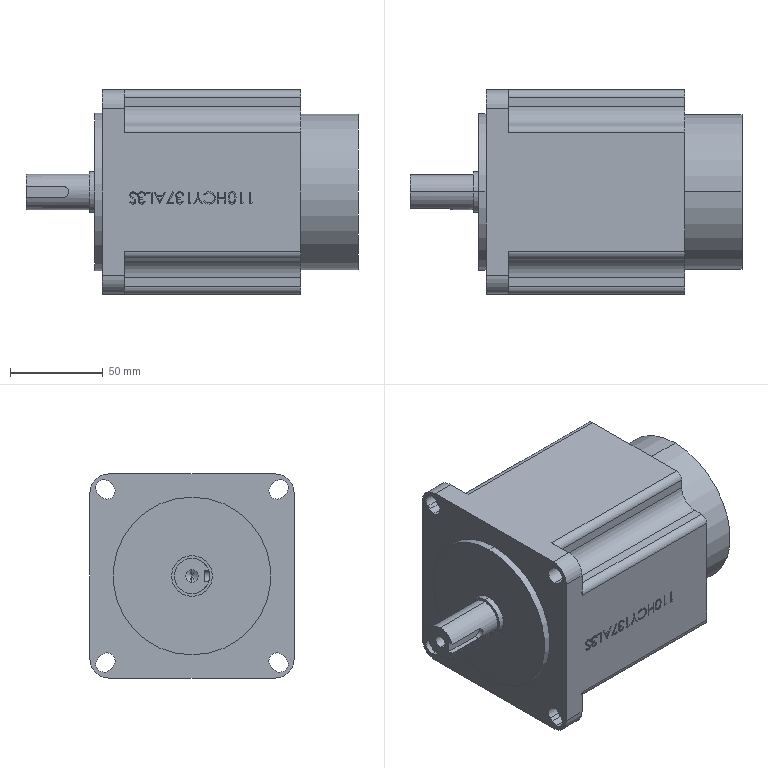Component | SolidWorks | ElectricalBoxAssembly2-1_StepperMotor-1 | 1 solid | 222 faces | box 179 x 110 x 110 mm | volume 1361866 mm3 | plane 120 | spline 61 | cylinder 39 | cone 2 | commonest cylinder face diameters 9 x12 20 x8 8 x8 6.8 x2 19 x2 22 x2 84 x2 85 x2
build123d program:
from build123d import *

# Parameters (mm, degrees)
SKETCH1_W             = 110
SKETCH1_H             = 110
BOSS_EXTRUDE1_DEPTH   = 12
SKETCH3_R             = 42.5
BOSS_EXTRUDE2_DEPTH   = 4
SKETCH4_R             = 9.5
BOSS_EXTRUDE3_DEPTH   = 37
CUT_EXTRUDE1_DEPTH    = 88.926
BOSS_EXTRUDE4_DEPTH   = 95
FILLET1_R             = 10
CUT_EXTRUDE2_DEPTH    = 3
SKETCH9_R             = 42
BOSS_EXTRUDE5_DEPTH   = 31
CUT_EXTRUDE3_DEPTH    = 0.1
SKETCH11_R            = 11
BOSS_EXTRUDE6_DEPTH   = 3
M8_TAPPED_HOLE1_D     = 6.8
M8_TAPPED_HOLE1_DEPTH = 15.4
M8_TAPPED_HOLE1_TIP   = 2.043


with BuildPart() as part:
    # Sketch1 → Boss-Extrude1 (new body)
    with BuildSketch(Plane(origin=(0, 0, 0), x_dir=(0, 0, -1), z_dir=(1, 0, 0))):
        Rectangle(SKETCH1_W, SKETCH1_H)
    extrude(amount=BOSS_EXTRUDE1_DEPTH)

    # Sketch3 → Boss-Extrude2 (add)
    with BuildSketch(Plane(origin=(12, 0, 0), x_dir=(0, 0, -1), z_dir=(1, 0, 0))):
        Circle(SKETCH3_R)
    extrude(amount=BOSS_EXTRUDE2_DEPTH)

    # Sketch4 → Boss-Extrude3 (add)
    with BuildSketch(Plane(origin=(16, 0, 0), x_dir=(0, 0, -1), z_dir=(1, 0, 0))):
        Circle(SKETCH4_R)
    extrude(amount=BOSS_EXTRUDE3_DEPTH)

    # Sketch5 → Cut-Extrude1 (cut, through all)
    with BuildSketch(Plane(origin=(12, 0, 0), x_dir=(0, 0, -1), z_dir=(1, 0, 0))):
        with BuildLine():
            Line((-44.194, 50.558), (-42.78, 49.144))
            ThreePointArc((-42.78, 49.144), (-42.78, 42.78), (-49.144, 42.78))
            Line((-49.144, 42.78), (-50.558, 44.194))
            ThreePointArc((-50.558, 44.194), (-50.558, 50.558), (-44.194, 50.558))
        make_face()
        with BuildLine():
            Line((50.558, 44.194), (49.144, 42.78))
            ThreePointArc((49.144, 42.78), (42.78, 42.78), (42.78, 49.144))
            Line((42.78, 49.144), (44.194, 50.558))
            ThreePointArc((44.194, 50.558), (50.558, 50.558), (50.558, 44.194))
        make_face()
        with BuildLine():
            Line((44.194, -50.558), (42.78, -49.144))
            ThreePointArc((42.78, -49.144), (42.78, -42.78), (49.144, -42.78))
            Line((49.144, -42.78), (50.558, -44.194))
            ThreePointArc((50.558, -44.194), (50.558, -50.558), (44.194, -50.558))
        make_face()
        with BuildLine():
            Line((-50.558, -44.194), (-49.144, -42.78))
            ThreePointArc((-49.144, -42.78), (-42.78, -42.78), (-42.78, -49.144))
            Line((-42.78, -49.144), (-44.194, -50.558))
            ThreePointArc((-44.194, -50.558), (-50.558, -50.558), (-50.558, -44.194))
        make_face()
    extrude(amount=-CUT_EXTRUDE1_DEPTH, mode=Mode.SUBTRACT)

    # Sketch6 → Boss-Extrude4 (add)
    with BuildSketch(Plane.ZY):
        with BuildLine():
            Line((31.962, -55), (-31.962, -55))
            ThreePointArc((-31.962, -55), (-34.79, -53.828), (-35.962, -51))
            Line((-35.962, -51), (-35.962, -45.962))
            ThreePointArc((-35.962, -45.962), (-38.891, -38.891), (-45.962, -35.962))
            Line((-45.962, -35.962), (-51, -35.962))
            ThreePointArc((-51, -35.962), (-53.828, -34.79), (-55, -31.962))
            Line((-55, -31.962), (-55, 31.962))
            ThreePointArc((-55, 31.962), (-53.828, 34.79), (-51, 35.962))
            Line((-51, 35.962), (-45.962, 35.962))
            ThreePointArc((-45.962, 35.962), (-38.891, 38.891), (-35.962, 45.962))
            Line((-35.962, 45.962), (-35.962, 51))
            ThreePointArc((-35.962, 51), (-34.79, 53.828), (-31.962, 55))
            Line((-31.962, 55), (31.962, 55))
            ThreePointArc((31.962, 55), (34.79, 53.828), (35.962, 51))
            Line((35.962, 51), (35.962, 45.962))
            ThreePointArc((35.962, 45.962), (38.891, 38.891), (45.962, 35.962))
            Line((45.962, 35.962), (51, 35.962))
            ThreePointArc((51, 35.962), (53.828, 34.79), (55, 31.962))
            Line((55, 31.962), (55, -31.962))
            ThreePointArc((55, -31.962), (53.828, -34.79), (51, -35.962))
            Line((51, -35.962), (45.962, -35.962))
            ThreePointArc((45.962, -35.962), (38.891, -38.891), (35.962, -45.962))
            Line((35.962, -45.962), (35.962, -51))
            ThreePointArc((35.962, -51), (34.79, -53.828), (31.962, -55))
        make_face()
    extrude(amount=BOSS_EXTRUDE4_DEPTH)

    # Fillet1
    fillet1_edges = [part.edges().sort_by_distance(p)[0] for p in [
        (6, -55, -55),
        (6, -55, 55),
        (6, 55, 55),
        (6, 55, -55),
    ]]
    fillet(fillet1_edges, radius=FILLET1_R)

    # Sketch7 → Cut-Extrude2 (cut)
    with BuildSketch(Plane(origin=(0, 9.5, 0), x_dir=(1, 0, 0), z_dir=(0, 1, 0))):
        with BuildLine():
            Line((73, -3), (33, -3))
            ThreePointArc((33, -3), (30, 0), (33, 3))
            Line((33, 3), (73, 3))
            ThreePointArc((73, 3), (76, 0), (73, -3))
        make_face()
    extrude(amount=-CUT_EXTRUDE2_DEPTH, mode=Mode.SUBTRACT)

    # Sketch9 → Boss-Extrude5 (add)
    with BuildSketch(Plane.ZY.offset(95)):
        Circle(SKETCH9_R)
    extrude(amount=BOSS_EXTRUDE5_DEPTH)

    # Sketch10 → Cut-Extrude3 (cut)
    # profile 1 of 13: a face of its own
    with BuildSketch(Plane(origin=(0, 55, 0), x_dir=(1, 0, 0), z_dir=(0, 1, 0))):
        Polygon((-68.662, 6.35), (-67.488, 6.35), (-67.488, 0), (-68.058, 0), (-68.058, 5.699), (-69.035, 5.699), align=None)
    # profile 2 of 13: a face of its own
    with BuildSketch(Plane(origin=(0, 55, 0), x_dir=(1, 0, 0), z_dir=(0, 1, 0))):
        Polygon((-63.778, 6.35), (-62.604, 6.35), (-62.604, 0), (-63.174, 0), (-63.174, 5.699), (-64.15, 5.699), align=None)
    # profile 3 of 13: a face of its own
    with BuildSketch(Plane(origin=(0, 55, 0), x_dir=(1, 0, 0), z_dir=(0, 1, 0))):
        with BuildLine():
            add(Edge.make_bspline(
                [(-60.243, 3.172), (-60.242, 3.274), (-60.241, 3.472), (-60.228, 3.76), (-60.207, 4.03), (-60.178, 4.283), (-60.142, 4.517), (-60.094, 4.734), (-60.04, 4.933), (-59.978, 5.115), (-59.907, 5.283), (-59.83, 5.44), (-59.744, 5.585), (-59.653, 5.721), (-59.554, 5.846), (-59.45, 5.962), (-59.337, 6.065), (-59.218, 6.159), (-59.093, 6.242), (-58.965, 6.314), (-58.833, 6.376), (-58.697, 6.425), (-58.557, 6.465), (-58.415, 6.493), (-58.269, 6.51), (-58.17, 6.512), (-58.12, 6.513)],
                knots=[0, 0, 0, 0, 1.646, 3.198, 4.664, 6.031, 7.308, 8.502, 9.612, 10.642, 11.616, 12.558, 13.465, 14.35, 15.204, 16.04, 16.86, 17.68, 18.487, 19.282, 20.062, 20.843, 21.62, 22.403, 23.19, 24, 24, 24, 24], degree=3))
            add(Edge.make_bspline(
                [(-58.12, 6.513), (-58.069, 6.512), (-57.969, 6.51), (-57.82, 6.493), (-57.675, 6.465), (-57.534, 6.425), (-57.396, 6.376), (-57.262, 6.314), (-57.131, 6.242), (-57.005, 6.158), (-56.883, 6.063), (-56.768, 5.957), (-56.66, 5.839), (-56.557, 5.711), (-56.463, 5.571), (-56.373, 5.421), (-56.292, 5.258), (-56.215, 5.085), (-56.148, 4.898), (-56.087, 4.697), (-56.039, 4.48), (-55.998, 4.248), (-55.966, 4.001), (-55.944, 3.738), (-55.931, 3.46), (-55.929, 3.27), (-55.928, 3.172)],
                knots=[0, 0, 0, 0, 0.8109, 1.613, 2.397, 3.182, 3.964, 4.75, 5.552, 6.362, 7.182, 8.026, 8.879, 9.751, 10.658, 11.592, 12.561, 13.573, 14.631, 15.753, 16.941, 18.2, 19.532, 20.947, 22.433, 24, 24, 24, 24], degree=3))
            add(Edge.make_bspline(
                [(-55.928, 3.172), (-55.929, 3.075), (-55.931, 2.886), (-55.943, 2.609), (-55.967, 2.348), (-55.996, 2.102), (-56.037, 1.871), (-56.087, 1.656), (-56.143, 1.455), (-56.211, 1.269), (-56.287, 1.097), (-56.368, 0.9359), (-56.456, 0.785), (-56.551, 0.6453), (-56.653, 0.5158), (-56.763, 0.3988), (-56.879, 0.2914), (-57.001, 0.1959), (-57.129, 0.1123), (-57.259, 0.03752), (-57.395, -0.02277), (-57.533, -0.07454), (-57.674, -0.1141), (-57.82, -0.1414), (-57.969, -0.1606), (-58.069, -0.1621), (-58.12, -0.1628)],
                knots=[0, 0, 0, 0, 1.562, 3.043, 4.452, 5.778, 7.032, 8.214, 9.334, 10.387, 11.391, 12.355, 13.287, 14.194, 15.073, 15.931, 16.776, 17.606, 18.423, 19.229, 20.022, 20.808, 21.593, 22.385, 23.188, 24, 24, 24, 24], degree=3))
            add(Edge.make_bspline(
                [(-58.12, -0.1628), (-58.17, -0.162), (-58.269, -0.1603), (-58.415, -0.143), (-58.557, -0.1153), (-58.695, -0.07644), (-58.831, -0.02888), (-58.962, 0.03309), (-59.089, 0.1044), (-59.213, 0.1857), (-59.331, 0.2788), (-59.444, 0.3818), (-59.548, 0.4973), (-59.646, 0.6233), (-59.738, 0.7588), (-59.823, 0.9056), (-59.902, 1.063), (-59.974, 1.233), (-60.038, 1.416), (-60.094, 1.616), (-60.138, 1.834), (-60.176, 2.068), (-60.207, 2.32), (-60.228, 2.589), (-60.241, 2.875), (-60.242, 3.072), (-60.243, 3.172)],
                knots=[0, 0, 0, 0, 0.8109, 1.599, 2.383, 3.153, 3.926, 4.706, 5.494, 6.292, 7.104, 7.925, 8.761, 9.623, 10.503, 11.417, 12.369, 13.354, 14.394, 15.514, 16.714, 17.995, 19.358, 20.818, 22.365, 24, 24, 24, 24], degree=3))
        make_face()
        with BuildLine():
            add(Edge.make_bspline(
                [(-59.673, 3.175), (-59.673, 3.09), (-59.672, 2.926), (-59.661, 2.686), (-59.646, 2.463), (-59.627, 2.256), (-59.598, 2.065), (-59.566, 1.89), (-59.527, 1.73), (-59.481, 1.586), (-59.428, 1.454), (-59.371, 1.331), (-59.309, 1.216), (-59.24, 1.11), (-59.164, 1.012), (-59.085, 0.9213), (-58.997, 0.84), (-58.877, 0.7425), (-58.717, 0.6418), (-58.517, 0.5541), (-58.31, 0.499), (-58.171, 0.492), (-58.101, 0.4885)],
                knots=[0, 0, 0, 0, 1.459, 2.832, 4.119, 5.306, 6.412, 7.436, 8.376, 9.234, 10.043, 10.816, 11.564, 12.286, 12.994, 13.686, 14.367, 15.042, 16.353, 17.594, 18.799, 20, 20, 20, 20], degree=3))
            add(Edge.make_bspline(
                [(-58.101, 0.4885), (-58.03, 0.4914), (-57.89, 0.4972), (-57.685, 0.553), (-57.485, 0.6373), (-57.329, 0.737), (-57.21, 0.832), (-57.125, 0.9129), (-57.047, 1.004), (-56.973, 1.101), (-56.905, 1.208), (-56.843, 1.323), (-56.787, 1.448), (-56.755, 1.534), (-56.738, 1.579)],
                knots=[0, 0, 0, 0, 1.354, 2.705, 4.075, 5.516, 6.261, 7.007, 7.778, 8.567, 9.372, 10.217, 11.089, 12, 12, 12, 12], degree=3))
            add(Edge.make_bspline(
                [(-56.738, 1.579), (-56.719, 1.635), (-56.68, 1.75), (-56.63, 1.929), (-56.591, 2.116), (-56.555, 2.311), (-56.531, 2.515), (-56.512, 2.727), (-56.5, 2.948), (-56.499, 3.099), (-56.498, 3.175)],
                knots=[0, 0, 0, 0, 0.8847, 1.796, 2.74, 3.715, 4.726, 5.778, 6.871, 8, 8, 8, 8], degree=3))
            add(Edge.make_bspline(
                [(-56.498, 3.175), (-56.499, 3.251), (-56.501, 3.401), (-56.508, 3.619), (-56.528, 3.827), (-56.549, 4.025), (-56.581, 4.211), (-56.615, 4.388), (-56.66, 4.553), (-56.709, 4.709), (-56.765, 4.853), (-56.827, 4.988), (-56.892, 5.113), (-56.964, 5.227), (-57.04, 5.333), (-57.123, 5.426), (-57.209, 5.511), (-57.331, 5.608), (-57.489, 5.707), (-57.687, 5.798), (-57.892, 5.85), (-58.031, 5.858), (-58.101, 5.862)],
                knots=[0, 0, 0, 0, 1.314, 2.57, 3.764, 4.902, 5.989, 7.016, 7.999, 8.933, 9.825, 10.668, 11.477, 12.251, 12.992, 13.711, 14.402, 15.077, 16.379, 17.61, 18.806, 20, 20, 20, 20], degree=3))
            add(Edge.make_bspline(
                [(-58.101, 5.862), (-58.171, 5.858), (-58.311, 5.85), (-58.519, 5.798), (-58.718, 5.708), (-58.876, 5.608), (-58.998, 5.513), (-59.083, 5.431), (-59.163, 5.341), (-59.237, 5.242), (-59.306, 5.136), (-59.37, 5.022), (-59.427, 4.898), (-59.48, 4.767), (-59.526, 4.622), (-59.564, 4.463), (-59.6, 4.288), (-59.625, 4.096), (-59.647, 3.889), (-59.661, 3.665), (-59.672, 3.426), (-59.673, 3.26), (-59.673, 3.175)],
                knots=[0, 0, 0, 0, 1.208, 2.418, 3.655, 4.956, 5.626, 6.302, 6.994, 7.697, 8.419, 9.17, 9.943, 10.752, 11.61, 12.549, 13.568, 14.68, 15.875, 17.154, 18.534, 20, 20, 20, 20], degree=3))
        make_face(mode=Mode.SUBTRACT)
    # profile 4 of 13: a face of its own
    with BuildSketch(Plane(origin=(0, 55, 0), x_dir=(1, 0, 0), z_dir=(0, 1, 0))):
        Polygon((-54.788, 6.35), (-54.218, 6.35), (-54.218, 3.745), (-50.962, 3.745), (-50.962, 6.35), (-50.392, 6.35), (-50.392, 0), (-50.962, 0), (-50.962, 3.094), (-54.218, 3.094), (-54.218, 0), (-54.788, 0), align=None)
    # profile 5 of 13: a face of its own
    with BuildSketch(Plane(origin=(0, 55, 0), x_dir=(1, 0, 0), z_dir=(0, 1, 0))):
        with BuildLine():
            Line((-42.902, 5.185), (-43.401, 4.803))
            add(Edge.make_bspline(
                [(-43.401, 4.803), (-43.437, 4.846), (-43.507, 4.93), (-43.621, 5.048), (-43.739, 5.159), (-43.863, 5.263), (-43.993, 5.356), (-44.127, 5.444), (-44.267, 5.522), (-44.461, 5.617), (-44.714, 5.717), (-45.033, 5.8), (-45.366, 5.853), (-45.593, 5.859), (-45.708, 5.862)],
                knots=[0, 0, 0, 0, 0.758, 1.506, 2.245, 2.98, 3.712, 4.438, 5.172, 5.909, 7.394, 8.89, 10.418, 12, 12, 12, 12], degree=3))
            add(Edge.make_bspline(
                [(-45.708, 5.862), (-45.772, 5.861), (-45.899, 5.859), (-46.087, 5.84), (-46.271, 5.813), (-46.452, 5.773), (-46.629, 5.722), (-46.804, 5.662), (-46.973, 5.586), (-47.139, 5.504), (-47.298, 5.41), (-47.449, 5.308), (-47.591, 5.198), (-47.723, 5.081), (-47.847, 4.956), (-47.961, 4.823), (-48.064, 4.682), (-48.16, 4.534), (-48.246, 4.381), (-48.317, 4.221), (-48.381, 4.058), (-48.431, 3.889), (-48.471, 3.715), (-48.498, 3.537), (-48.517, 3.355), (-48.519, 3.231), (-48.52, 3.169)],
                knots=[0, 0, 0, 0, 1.055, 2.1, 3.131, 4.146, 5.17, 6.184, 7.204, 8.235, 9.262, 10.264, 11.252, 12.228, 13.197, 14.16, 15.13, 16.101, 17.073, 18.039, 19.003, 19.979, 20.96, 21.949, 22.966, 24, 24, 24, 24], degree=3))
            add(Edge.make_bspline(
                [(-48.52, 3.169), (-48.517, 3.075), (-48.513, 2.891), (-48.473, 2.621), (-48.412, 2.362), (-48.321, 2.116), (-48.209, 1.881), (-48.067, 1.659), (-47.902, 1.448), (-47.713, 1.252), (-47.506, 1.073), (-47.283, 0.9159), (-47.046, 0.7847), (-46.796, 0.6756), (-46.533, 0.5916), (-46.257, 0.5326), (-45.967, 0.494), (-45.77, 0.4903), (-45.669, 0.4885)],
                knots=[0, 0, 0, 0, 1.029, 2.021, 2.988, 3.938, 4.889, 5.847, 6.821, 7.821, 8.828, 9.823, 10.808, 11.797, 12.804, 13.832, 14.897, 16, 16, 16, 16], degree=3))
            add(Edge.make_bspline(
                [(-45.669, 0.4885), (-45.558, 0.4915), (-45.34, 0.4976), (-45.02, 0.5486), (-44.714, 0.6315), (-44.421, 0.7474), (-44.143, 0.8981), (-43.879, 1.081), (-43.628, 1.297), (-43.478, 1.462), (-43.401, 1.547)],
                knots=[0, 0, 0, 0, 1.028, 2.024, 2.998, 3.968, 4.937, 5.927, 6.942, 8, 8, 8, 8], degree=3))
            Line((-43.401, 1.547), (-42.902, 1.169))
            add(Edge.make_bspline(
                [(-42.902, 1.169), (-42.942, 1.117), (-43.023, 1.014), (-43.152, 0.8683), (-43.289, 0.7313), (-43.433, 0.6041), (-43.584, 0.484), (-43.744, 0.3746), (-43.911, 0.2743), (-44.084, 0.1825), (-44.263, 0.101), (-44.448, 0.03121), (-44.638, -0.02889), (-44.833, -0.07833), (-45.034, -0.1169), (-45.24, -0.1427), (-45.451, -0.1604), (-45.593, -0.162), (-45.665, -0.1628)],
                knots=[0, 0, 0, 0, 0.9868, 1.969, 2.936, 3.9, 4.868, 5.838, 6.815, 7.798, 8.788, 9.778, 10.776, 11.791, 12.813, 13.856, 14.914, 16, 16, 16, 16], degree=3))
            add(Edge.make_bspline(
                [(-45.665, -0.1628), (-45.734, -0.1623), (-45.869, -0.1614), (-46.068, -0.1462), (-46.262, -0.1254), (-46.45, -0.09413), (-46.634, -0.05722), (-46.811, -0.00774), (-46.983, 0.04769), (-47.15, 0.1128), (-47.312, 0.1863), (-47.467, 0.2694), (-47.617, 0.3614), (-47.763, 0.4602), (-47.902, 0.569), (-48.035, 0.6863), (-48.164, 0.8117), (-48.244, 0.9022), (-48.284, 0.9477)],
                knots=[0, 0, 0, 0, 1.115, 2.204, 3.263, 4.3, 5.319, 6.316, 7.299, 8.272, 9.238, 10.195, 11.152, 12.108, 13.065, 14.031, 15.01, 16, 16, 16, 16], degree=3))
            add(Edge.make_bspline(
                [(-48.284, 0.9477), (-48.349, 1.027), (-48.476, 1.184), (-48.64, 1.438), (-48.78, 1.704), (-48.893, 1.982), (-48.982, 2.273), (-49.043, 2.575), (-49.083, 2.889), (-49.087, 3.103), (-49.09, 3.212)],
                knots=[0, 0, 0, 0, 0.9946, 1.977, 2.95, 3.926, 4.909, 5.912, 6.938, 8, 8, 8, 8], degree=3))
            add(Edge.make_bspline(
                [(-49.09, 3.212), (-49.087, 3.326), (-49.081, 3.551), (-49.034, 3.881), (-48.958, 4.197), (-48.85, 4.498), (-48.714, 4.787), (-48.545, 5.06), (-48.346, 5.321), (-48.118, 5.564), (-47.869, 5.786), (-47.602, 5.982), (-47.317, 6.145), (-47.019, 6.281), (-46.704, 6.385), (-46.374, 6.459), (-46.028, 6.504), (-45.793, 6.51), (-45.673, 6.513)],
                knots=[0, 0, 0, 0, 1.033, 2.032, 3.007, 3.968, 4.924, 5.892, 6.872, 7.884, 8.9, 9.891, 10.874, 11.86, 12.855, 13.869, 14.917, 16, 16, 16, 16], degree=3))
            add(Edge.make_bspline(
                [(-45.673, 6.513), (-45.6, 6.512), (-45.455, 6.51), (-45.242, 6.493), (-45.034, 6.465), (-44.831, 6.427), (-44.633, 6.379), (-44.441, 6.317), (-44.254, 6.247), (-44.073, 6.165), (-43.899, 6.073), (-43.732, 5.973), (-43.574, 5.864), (-43.422, 5.746), (-43.28, 5.618), (-43.144, 5.484), (-43.019, 5.338), (-42.941, 5.236), (-42.902, 5.185)],
                knots=[0, 0, 0, 0, 1.097, 2.171, 3.219, 4.251, 5.268, 6.278, 7.281, 8.274, 9.261, 10.236, 11.203, 12.157, 13.114, 14.07, 15.032, 16, 16, 16, 16], degree=3))
        make_face()
    # profile 6 of 13: a face of its own
    with BuildSketch(Plane(origin=(0, 55, 0), x_dir=(1, 0, 0), z_dir=(0, 1, 0))):
        Polygon((-42.088, 6.35), (-41.436, 6.35), (-39.767, 3.621), (-38.1, 6.35), (-37.448, 6.35), (-39.483, 3.019), (-39.483, 0), (-40.053, 0), (-40.053, 3.019), align=None)
    # profile 7 of 13: a face of its own
    with BuildSketch(Plane(origin=(0, 55, 0), x_dir=(1, 0, 0), z_dir=(0, 1, 0))):
        Polygon((-35.528, 6.35), (-34.354, 6.35), (-34.354, 0), (-34.924, 0), (-34.924, 5.699), (-35.901, 5.699), align=None)
    # profile 8 of 13: a face of its own
    with BuildSketch(Plane(origin=(0, 55, 0), x_dir=(1, 0, 0), z_dir=(0, 1, 0))):
        with BuildLine():
            Line((-31.179, 4.885), (-31.749, 4.885))
            add(Edge.make_bspline(
                [(-31.749, 4.885), (-31.734, 4.949), (-31.704, 5.073), (-31.641, 5.252), (-31.572, 5.421), (-31.49, 5.577), (-31.4, 5.724), (-31.297, 5.857), (-31.186, 5.982), (-31.063, 6.092), (-30.934, 6.191), (-30.797, 6.277), (-30.655, 6.35), (-30.507, 6.41), (-30.352, 6.455), (-30.193, 6.488), (-30.028, 6.51), (-29.916, 6.512), (-29.859, 6.513)],
                knots=[0, 0, 0, 0, 1.162, 2.272, 3.344, 4.383, 5.39, 6.38, 7.362, 8.333, 9.296, 10.242, 11.178, 12.116, 13.063, 14.02, 14.995, 16, 16, 16, 16], degree=3))
            add(Edge.make_bspline(
                [(-29.859, 6.513), (-29.776, 6.51), (-29.612, 6.505), (-29.371, 6.46), (-29.139, 6.389), (-28.918, 6.29), (-28.712, 6.168), (-28.53, 6.023), (-28.372, 5.857), (-28.24, 5.675), (-28.136, 5.479), (-28.06, 5.278), (-28.013, 5.072), (-28.007, 4.933), (-28.004, 4.863)],
                knots=[0, 0, 0, 0, 1.083, 2.142, 3.193, 4.256, 5.303, 6.309, 7.297, 8.282, 9.25, 10.18, 11.088, 12, 12, 12, 12], degree=3))
            add(Edge.make_bspline(
                [(-28.004, 4.863), (-28.006, 4.796), (-28.011, 4.664), (-28.046, 4.473), (-28.105, 4.292), (-28.186, 4.121), (-28.292, 3.962), (-28.42, 3.814), (-28.572, 3.676), (-28.687, 3.597), (-28.746, 3.557)],
                knots=[0, 0, 0, 0, 1.025, 2.005, 2.965, 3.921, 4.883, 5.875, 6.906, 8, 8, 8, 8], degree=3))
            add(Edge.make_bspline(
                [(-28.746, 3.557), (-28.678, 3.524), (-28.545, 3.459), (-28.362, 3.333), (-28.196, 3.186), (-28.104, 3.072), (-28.058, 3.015)],
                knots=[0, 0, 0, 0, 1.016, 2.012, 3.001, 4, 4, 4, 4], degree=3))
            add(Edge.make_bspline(
                [(-28.058, 3.015), (-28.027, 2.973), (-27.967, 2.89), (-27.892, 2.756), (-27.824, 2.622), (-27.771, 2.482), (-27.73, 2.338), (-27.701, 2.191), (-27.683, 2.04), (-27.68, 1.938), (-27.679, 1.886)],
                knots=[0, 0, 0, 0, 1.025, 2.033, 3.025, 4.014, 4.992, 5.977, 6.983, 8, 8, 8, 8], degree=3))
            add(Edge.make_bspline(
                [(-27.679, 1.886), (-27.682, 1.798), (-27.688, 1.62), (-27.746, 1.358), (-27.836, 1.102), (-27.964, 0.8567), (-28.12, 0.6274), (-28.305, 0.4222), (-28.518, 0.2459), (-28.756, 0.09856), (-29.013, -0.01922), (-29.288, -0.101), (-29.577, -0.1542), (-29.775, -0.1599), (-29.875, -0.1628)],
                knots=[0, 0, 0, 0, 0.9558, 1.907, 2.875, 3.871, 4.872, 5.851, 6.836, 7.836, 8.849, 9.87, 10.917, 12, 12, 12, 12], degree=3))
            add(Edge.make_bspline(
                [(-29.875, -0.1628), (-29.943, -0.1612), (-30.077, -0.1581), (-30.273, -0.137), (-30.461, -0.09826), (-30.64, -0.04618), (-30.81, 0.01984), (-30.971, 0.1021), (-31.124, 0.1988), (-31.268, 0.3112), (-31.402, 0.4368), (-31.523, 0.5781), (-31.633, 0.7323), (-31.729, 0.9013), (-31.816, 1.083), (-31.887, 1.279), (-31.949, 1.489), (-31.978, 1.635), (-31.993, 1.71)],
                knots=[0, 0, 0, 0, 1.049, 2.063, 3.046, 4.001, 4.937, 5.862, 6.793, 7.731, 8.676, 9.628, 10.6, 11.598, 12.626, 13.702, 14.821, 16, 16, 16, 16], degree=3))
            Line((-31.993, 1.71), (-31.424, 1.71))
            add(Edge.make_bspline(
                [(-31.424, 1.71), (-31.409, 1.661), (-31.38, 1.566), (-31.331, 1.429), (-31.275, 1.303), (-31.215, 1.188), (-31.151, 1.083), (-31.081, 0.9891), (-31.008, 0.9036), (-30.953, 0.8555), (-30.926, 0.8319)],
                knots=[0, 0, 0, 0, 1.198, 2.331, 3.408, 4.417, 5.372, 6.289, 7.163, 8, 8, 8, 8], degree=3))
            add(Edge.make_bspline(
                [(-30.926, 0.8319), (-30.891, 0.8045), (-30.82, 0.7498), (-30.704, 0.6799), (-30.582, 0.6194), (-30.452, 0.5731), (-30.316, 0.534), (-30.172, 0.5084), (-30.021, 0.4908), (-29.918, 0.4893), (-29.865, 0.4885)],
                knots=[0, 0, 0, 0, 0.9462, 1.889, 2.845, 3.807, 4.801, 5.829, 6.891, 8, 8, 8, 8], degree=3))
            add(Edge.make_bspline(
                [(-29.865, 0.4885), (-29.806, 0.4896), (-29.69, 0.4918), (-29.52, 0.5119), (-29.359, 0.5411), (-29.208, 0.5863), (-29.064, 0.6422), (-28.931, 0.7123), (-28.806, 0.7946), (-28.691, 0.8881), (-28.588, 0.9904), (-28.497, 1.097), (-28.42, 1.209), (-28.357, 1.325), (-28.308, 1.446), (-28.275, 1.571), (-28.251, 1.7), (-28.249, 1.788), (-28.249, 1.832)],
                knots=[0, 0, 0, 0, 1.217, 2.38, 3.494, 4.572, 5.61, 6.639, 7.649, 8.668, 9.67, 10.625, 11.543, 12.441, 13.322, 14.205, 15.095, 16, 16, 16, 16], degree=3))
            add(Edge.make_bspline(
                [(-28.249, 1.832), (-28.251, 1.891), (-28.257, 2.009), (-28.299, 2.183), (-28.369, 2.35), (-28.466, 2.508), (-28.585, 2.655), (-28.723, 2.785), (-28.883, 2.893), (-29.03, 2.968), (-29.16, 3.019), (-29.271, 3.053), (-29.396, 3.081), (-29.533, 3.108), (-29.682, 3.131), (-29.844, 3.15), (-30.019, 3.165), (-30.14, 3.172), (-30.202, 3.175)],
                knots=[0, 0, 0, 0, 1.071, 2.136, 3.217, 4.34, 5.486, 6.621, 7.776, 8.964, 9.598, 10.305, 11.07, 11.915, 12.824, 13.806, 14.869, 16, 16, 16, 16], degree=3))
            Line((-30.202, 3.175), (-30.202, 3.826))
            add(Edge.make_bspline(
                [(-30.202, 3.826), (-30.124, 3.828), (-29.97, 3.83), (-29.745, 3.862), (-29.53, 3.905), (-29.33, 3.972), (-29.147, 4.05), (-28.989, 4.141), (-28.857, 4.241), (-28.752, 4.353), (-28.673, 4.474), (-28.615, 4.599), (-28.581, 4.731), (-28.576, 4.82), (-28.574, 4.866)],
                knots=[0, 0, 0, 0, 1.322, 2.589, 3.816, 5.011, 6.14, 7.154, 8.075, 8.924, 9.728, 10.489, 11.24, 12, 12, 12, 12], degree=3))
            add(Edge.make_bspline(
                [(-28.574, 4.866), (-28.575, 4.899), (-28.576, 4.965), (-28.595, 5.061), (-28.624, 5.154), (-28.663, 5.245), (-28.715, 5.331), (-28.777, 5.414), (-28.852, 5.493), (-28.937, 5.567), (-29.028, 5.637), (-29.128, 5.697), (-29.234, 5.748), (-29.346, 5.79), (-29.464, 5.821), (-29.588, 5.844), (-29.718, 5.858), (-29.806, 5.86), (-29.851, 5.862)],
                knots=[0, 0, 0, 0, 0.8844, 1.759, 2.612, 3.489, 4.373, 5.295, 6.256, 7.267, 8.302, 9.333, 10.376, 11.44, 12.52, 13.637, 14.799, 16, 16, 16, 16], degree=3))
            add(Edge.make_bspline(
                [(-29.851, 5.862), (-29.924, 5.859), (-30.065, 5.854), (-30.268, 5.811), (-30.458, 5.742), (-30.602, 5.66), (-30.709, 5.579), (-30.786, 5.508), (-30.86, 5.429), (-30.929, 5.337), (-30.999, 5.239), (-31.062, 5.13), (-31.123, 5.011), (-31.16, 4.928), (-31.179, 4.885)],
                knots=[0, 0, 0, 0, 1.473, 2.876, 4.222, 5.565, 6.25, 6.953, 7.687, 8.464, 9.284, 10.136, 11.041, 12, 12, 12, 12], degree=3))
        make_face()
    # profile 9 of 13: a face of its own
    with BuildSketch(Plane(origin=(0, 55, 0), x_dir=(1, 0, 0), z_dir=(0, 1, 0))):
        Polygon((-26.702, 6.35), (-22.794, 6.35), (-26.132, -0.1628), (-26.624, 0.1081), (-23.758, 5.699), (-26.702, 5.699), align=None)
    # profile 10 of 13: a face of its own
    with BuildSketch(Plane(origin=(0, 55, 0), x_dir=(1, 0, 0), z_dir=(0, 1, 0))):
        Polygon((-19.049, 6.35), (-16.118, 0), (-16.738, 0), (-17.677, 2.035), (-20.555, 2.035), (-21.521, 0), (-22.143, 0), (-19.131, 6.35), align=None)
        Polygon((-19.096, 5.112), (-20.246, 2.687), (-17.977, 2.687), align=None, mode=Mode.SUBTRACT)
    # profile 11 of 13: a face of its own
    with BuildSketch(Plane(origin=(0, 55, 0), x_dir=(1, 0, 0), z_dir=(0, 1, 0))):
        Polygon((-14.979, 6.35), (-14.409, 6.35), (-14.409, 0.6513), (-11.966, 0.6513), (-11.966, 0), (-14.979, 0), align=None)
    # profile 12 of 13: a face of its own
    with BuildSketch(Plane(origin=(0, 55, 0), x_dir=(1, 0, 0), z_dir=(0, 1, 0))):
        with BuildLine():
            Line((-10.664, 4.885), (-11.234, 4.885))
            add(Edge.make_bspline(
                [(-11.234, 4.885), (-11.218, 4.949), (-11.188, 5.073), (-11.125, 5.252), (-11.057, 5.421), (-10.974, 5.577), (-10.884, 5.724), (-10.782, 5.857), (-10.67, 5.982), (-10.547, 6.092), (-10.418, 6.191), (-10.281, 6.277), (-10.139, 6.35), (-9.991, 6.41), (-9.837, 6.455), (-9.677, 6.488), (-9.512, 6.51), (-9.4, 6.512), (-9.344, 6.513)],
                knots=[0, 0, 0, 0, 1.162, 2.272, 3.344, 4.383, 5.39, 6.38, 7.362, 8.333, 9.296, 10.242, 11.178, 12.116, 13.063, 14.02, 14.995, 16, 16, 16, 16], degree=3))
            add(Edge.make_bspline(
                [(-9.344, 6.513), (-9.261, 6.51), (-9.097, 6.505), (-8.856, 6.46), (-8.624, 6.389), (-8.402, 6.29), (-8.197, 6.168), (-8.014, 6.023), (-7.857, 5.857), (-7.724, 5.675), (-7.621, 5.479), (-7.544, 5.278), (-7.498, 5.072), (-7.492, 4.933), (-7.489, 4.863)],
                knots=[0, 0, 0, 0, 1.083, 2.142, 3.193, 4.256, 5.303, 6.309, 7.297, 8.282, 9.25, 10.18, 11.088, 12, 12, 12, 12], degree=3))
            add(Edge.make_bspline(
                [(-7.489, 4.863), (-7.491, 4.796), (-7.495, 4.664), (-7.53, 4.473), (-7.589, 4.292), (-7.671, 4.121), (-7.777, 3.962), (-7.905, 3.814), (-8.057, 3.676), (-8.171, 3.597), (-8.231, 3.557)],
                knots=[0, 0, 0, 0, 1.025, 2.005, 2.965, 3.921, 4.883, 5.875, 6.906, 8, 8, 8, 8], degree=3))
            add(Edge.make_bspline(
                [(-8.231, 3.557), (-8.163, 3.524), (-8.029, 3.459), (-7.847, 3.333), (-7.681, 3.186), (-7.589, 3.072), (-7.542, 3.015)],
                knots=[0, 0, 0, 0, 1.016, 2.012, 3.001, 4, 4, 4, 4], degree=3))
            add(Edge.make_bspline(
                [(-7.542, 3.015), (-7.512, 2.973), (-7.451, 2.89), (-7.376, 2.756), (-7.308, 2.622), (-7.256, 2.482), (-7.215, 2.338), (-7.185, 2.191), (-7.167, 2.04), (-7.165, 1.938), (-7.163, 1.886)],
                knots=[0, 0, 0, 0, 1.025, 2.033, 3.025, 4.014, 4.992, 5.977, 6.983, 8, 8, 8, 8], degree=3))
            add(Edge.make_bspline(
                [(-7.163, 1.886), (-7.167, 1.798), (-7.173, 1.62), (-7.231, 1.358), (-7.321, 1.102), (-7.449, 0.8567), (-7.605, 0.6274), (-7.79, 0.4222), (-8.003, 0.2459), (-8.24, 0.09856), (-8.497, -0.01922), (-8.772, -0.101), (-9.061, -0.1542), (-9.259, -0.1599), (-9.36, -0.1628)],
                knots=[0, 0, 0, 0, 0.9558, 1.907, 2.875, 3.871, 4.872, 5.851, 6.836, 7.836, 8.849, 9.87, 10.917, 12, 12, 12, 12], degree=3))
            add(Edge.make_bspline(
                [(-9.36, -0.1628), (-9.428, -0.1612), (-9.562, -0.1581), (-9.758, -0.137), (-9.945, -0.09826), (-10.124, -0.04618), (-10.294, 0.01984), (-10.456, 0.1021), (-10.609, 0.1988), (-10.753, 0.3112), (-10.887, 0.4368), (-11.008, 0.5781), (-11.118, 0.7323), (-11.214, 0.9013), (-11.3, 1.083), (-11.371, 1.279), (-11.434, 1.489), (-11.463, 1.635), (-11.478, 1.71)],
                knots=[0, 0, 0, 0, 1.049, 2.063, 3.046, 4.001, 4.937, 5.862, 6.793, 7.731, 8.676, 9.628, 10.6, 11.598, 12.626, 13.702, 14.821, 16, 16, 16, 16], degree=3))
            Line((-11.478, 1.71), (-10.908, 1.71))
            add(Edge.make_bspline(
                [(-10.908, 1.71), (-10.893, 1.661), (-10.864, 1.566), (-10.815, 1.429), (-10.759, 1.303), (-10.699, 1.188), (-10.636, 1.083), (-10.565, 0.9891), (-10.493, 0.9036), (-10.438, 0.8555), (-10.411, 0.8319)],
                knots=[0, 0, 0, 0, 1.198, 2.331, 3.408, 4.417, 5.372, 6.289, 7.163, 8, 8, 8, 8], degree=3))
            add(Edge.make_bspline(
                [(-10.411, 0.8319), (-10.375, 0.8045), (-10.304, 0.7498), (-10.189, 0.6799), (-10.067, 0.6194), (-9.937, 0.5731), (-9.8, 0.534), (-9.656, 0.5084), (-9.506, 0.4908), (-9.403, 0.4893), (-9.35, 0.4885)],
                knots=[0, 0, 0, 0, 0.9462, 1.889, 2.845, 3.807, 4.801, 5.829, 6.891, 8, 8, 8, 8], degree=3))
            add(Edge.make_bspline(
                [(-9.35, 0.4885), (-9.29, 0.4896), (-9.174, 0.4918), (-9.005, 0.5119), (-8.843, 0.5411), (-8.692, 0.5863), (-8.549, 0.6422), (-8.416, 0.7123), (-8.291, 0.7946), (-8.176, 0.8881), (-8.073, 0.9904), (-7.982, 1.097), (-7.904, 1.209), (-7.842, 1.325), (-7.793, 1.446), (-7.759, 1.571), (-7.736, 1.7), (-7.734, 1.788), (-7.733, 1.832)],
                knots=[0, 0, 0, 0, 1.217, 2.38, 3.494, 4.572, 5.61, 6.639, 7.649, 8.668, 9.67, 10.625, 11.543, 12.441, 13.322, 14.205, 15.095, 16, 16, 16, 16], degree=3))
            add(Edge.make_bspline(
                [(-7.733, 1.832), (-7.736, 1.891), (-7.741, 2.009), (-7.784, 2.183), (-7.853, 2.35), (-7.951, 2.508), (-8.069, 2.655), (-8.208, 2.785), (-8.367, 2.893), (-8.514, 2.968), (-8.645, 3.019), (-8.756, 3.053), (-8.881, 3.081), (-9.017, 3.108), (-9.167, 3.131), (-9.329, 3.15), (-9.504, 3.165), (-9.625, 3.172), (-9.687, 3.175)],
                knots=[0, 0, 0, 0, 1.071, 2.136, 3.217, 4.34, 5.486, 6.621, 7.776, 8.964, 9.598, 10.305, 11.07, 11.915, 12.824, 13.806, 14.869, 16, 16, 16, 16], degree=3))
            Line((-9.687, 3.175), (-9.687, 3.826))
            add(Edge.make_bspline(
                [(-9.687, 3.826), (-9.608, 3.828), (-9.455, 3.83), (-9.23, 3.862), (-9.015, 3.905), (-8.814, 3.972), (-8.632, 4.05), (-8.473, 4.141), (-8.341, 4.241), (-8.236, 4.353), (-8.157, 4.474), (-8.1, 4.599), (-8.066, 4.731), (-8.061, 4.82), (-8.059, 4.866)],
                knots=[0, 0, 0, 0, 1.322, 2.589, 3.816, 5.011, 6.14, 7.154, 8.075, 8.924, 9.728, 10.489, 11.24, 12, 12, 12, 12], degree=3))
            add(Edge.make_bspline(
                [(-8.059, 4.866), (-8.06, 4.899), (-8.061, 4.965), (-8.08, 5.061), (-8.108, 5.154), (-8.147, 5.245), (-8.199, 5.331), (-8.262, 5.414), (-8.336, 5.493), (-8.421, 5.567), (-8.513, 5.637), (-8.613, 5.697), (-8.719, 5.748), (-8.831, 5.79), (-8.949, 5.821), (-9.073, 5.844), (-9.202, 5.858), (-9.291, 5.86), (-9.336, 5.862)],
                knots=[0, 0, 0, 0, 0.8844, 1.759, 2.612, 3.489, 4.373, 5.295, 6.256, 7.267, 8.302, 9.333, 10.376, 11.44, 12.52, 13.637, 14.799, 16, 16, 16, 16], degree=3))
            add(Edge.make_bspline(
                [(-9.336, 5.862), (-9.408, 5.859), (-9.549, 5.854), (-9.753, 5.811), (-9.942, 5.742), (-10.087, 5.66), (-10.194, 5.579), (-10.27, 5.508), (-10.345, 5.429), (-10.414, 5.337), (-10.483, 5.239), (-10.546, 5.13), (-10.608, 5.011), (-10.645, 4.928), (-10.664, 4.885)],
                knots=[0, 0, 0, 0, 1.473, 2.876, 4.222, 5.565, 6.25, 6.953, 7.687, 8.464, 9.284, 10.136, 11.041, 12, 12, 12, 12], degree=3))
        make_face()
    # profile 13 of 13: a face of its own
    with BuildSketch(Plane(origin=(0, 55, 0), x_dir=(1, 0, 0), z_dir=(0, 1, 0))):
        with BuildLine():
            Line((-6.675, 1.225), (-6.138, 1.547))
            add(Edge.make_bspline(
                [(-6.138, 1.547), (-6.088, 1.463), (-5.992, 1.303), (-5.833, 1.087), (-5.668, 0.9028), (-5.495, 0.7525), (-5.317, 0.6341), (-5.132, 0.5503), (-4.94, 0.498), (-4.809, 0.4916), (-4.744, 0.4885)],
                knots=[0, 0, 0, 0, 1.272, 2.437, 3.508, 4.499, 5.419, 6.295, 7.149, 8, 8, 8, 8], degree=3))
            add(Edge.make_bspline(
                [(-4.744, 0.4885), (-4.688, 0.49), (-4.578, 0.4931), (-4.415, 0.5226), (-4.258, 0.568), (-4.108, 0.633), (-3.968, 0.7116), (-3.845, 0.8066), (-3.739, 0.9129), (-3.652, 1.032), (-3.586, 1.159), (-3.535, 1.29), (-3.506, 1.426), (-3.502, 1.518), (-3.5, 1.565)],
                knots=[0, 0, 0, 0, 1.095, 2.171, 3.241, 4.322, 5.38, 6.392, 7.366, 8.328, 9.273, 10.192, 11.088, 12, 12, 12, 12], degree=3))
            add(Edge.make_bspline(
                [(-3.5, 1.565), (-3.502, 1.617), (-3.508, 1.725), (-3.554, 1.884), (-3.626, 2.04), (-3.693, 2.138), (-3.727, 2.188)],
                knots=[0, 0, 0, 0, 0.9389, 1.909, 2.914, 4, 4, 4, 4], degree=3))
            add(Edge.make_bspline(
                [(-3.727, 2.188), (-3.756, 2.224), (-3.816, 2.301), (-3.918, 2.414), (-4.039, 2.532), (-4.173, 2.657), (-4.325, 2.784), (-4.492, 2.92), (-4.676, 3.059), (-4.806, 3.152), (-4.872, 3.2)],
                knots=[0, 0, 0, 0, 0.7222, 1.516, 2.394, 3.351, 4.387, 5.505, 6.713, 8, 8, 8, 8], degree=3))
            add(Edge.make_bspline(
                [(-4.872, 3.2), (-4.939, 3.248), (-5.067, 3.339), (-5.246, 3.474), (-5.405, 3.597), (-5.545, 3.711), (-5.666, 3.813), (-5.768, 3.904), (-5.848, 3.987), (-5.893, 4.04), (-5.913, 4.064)],
                knots=[0, 0, 0, 0, 1.452, 2.777, 3.965, 5.027, 5.964, 6.767, 7.446, 8, 8, 8, 8], degree=3))
            add(Edge.make_bspline(
                [(-5.913, 4.064), (-5.941, 4.102), (-5.996, 4.175), (-6.069, 4.29), (-6.131, 4.408), (-6.179, 4.528), (-6.22, 4.65), (-6.248, 4.775), (-6.265, 4.902), (-6.267, 4.988), (-6.268, 5.031)],
                knots=[0, 0, 0, 0, 1.068, 2.1, 3.106, 4.101, 5.07, 6.043, 7.02, 8, 8, 8, 8], degree=3))
            add(Edge.make_bspline(
                [(-6.268, 5.031), (-6.265, 5.098), (-6.261, 5.231), (-6.221, 5.425), (-6.159, 5.611), (-6.071, 5.785), (-5.958, 5.945), (-5.827, 6.091), (-5.672, 6.214), (-5.501, 6.322), (-5.314, 6.406), (-5.118, 6.469), (-4.913, 6.505), (-4.774, 6.51), (-4.703, 6.513)],
                knots=[0, 0, 0, 0, 1.005, 1.989, 2.955, 3.93, 4.906, 5.877, 6.857, 7.866, 8.892, 9.919, 10.944, 12, 12, 12, 12], degree=3))
            add(Edge.make_bspline(
                [(-4.703, 6.513), (-4.628, 6.51), (-4.48, 6.505), (-4.261, 6.46), (-4.05, 6.387), (-3.88, 6.303), (-3.748, 6.219), (-3.646, 6.143), (-3.544, 6.055), (-3.439, 5.956), (-3.334, 5.843), (-3.227, 5.719), (-3.118, 5.584), (-3.047, 5.487), (-3.011, 5.438)],
                knots=[0, 0, 0, 0, 1.287, 2.559, 3.826, 5.122, 5.804, 6.523, 7.3, 8.126, 9.008, 9.945, 10.946, 12, 12, 12, 12], degree=3))
            Line((-3.011, 5.438), (-3.527, 5.047))
            add(Edge.make_bspline(
                [(-3.527, 5.047), (-3.558, 5.088), (-3.618, 5.165), (-3.708, 5.273), (-3.794, 5.371), (-3.879, 5.457), (-3.957, 5.535), (-4.034, 5.601), (-4.107, 5.657), (-4.199, 5.716), (-4.314, 5.776), (-4.46, 5.826), (-4.611, 5.856), (-4.714, 5.86), (-4.767, 5.862)],
                knots=[0, 0, 0, 0, 1.182, 2.276, 3.29, 4.226, 5.078, 5.863, 6.582, 7.217, 8.414, 9.595, 10.783, 12, 12, 12, 12], degree=3))
            add(Edge.make_bspline(
                [(-4.767, 5.862), (-4.832, 5.859), (-4.959, 5.855), (-5.138, 5.809), (-5.3, 5.736), (-5.439, 5.634), (-5.555, 5.513), (-5.638, 5.373), (-5.689, 5.22), (-5.695, 5.112), (-5.698, 5.058)],
                knots=[0, 0, 0, 0, 1.145, 2.207, 3.219, 4.227, 5.203, 6.127, 7.046, 8, 8, 8, 8], degree=3))
            add(Edge.make_bspline(
                [(-5.698, 5.058), (-5.697, 5.024), (-5.696, 4.955), (-5.676, 4.855), (-5.65, 4.755), (-5.61, 4.655), (-5.554, 4.554), (-5.48, 4.451), (-5.388, 4.344), (-5.317, 4.274), (-5.279, 4.237)],
                knots=[0, 0, 0, 0, 0.8583, 1.718, 2.584, 3.473, 4.427, 5.489, 6.674, 8, 8, 8, 8], degree=3))
            add(Edge.make_bspline(
                [(-5.279, 4.237), (-5.265, 4.225), (-5.232, 4.195), (-5.172, 4.147), (-5.092, 4.088), (-4.995, 4.014), (-4.879, 3.928), (-4.744, 3.832), (-4.591, 3.722), (-4.483, 3.646), (-4.426, 3.605)],
                knots=[0, 0, 0, 0, 0.4208, 0.9996, 1.745, 2.668, 3.75, 5, 6.413, 8, 8, 8, 8], degree=3))
            add(Edge.make_bspline(
                [(-4.426, 3.605), (-4.357, 3.555), (-4.223, 3.458), (-4.034, 3.312), (-3.861, 3.169), (-3.706, 3.031), (-3.567, 2.897), (-3.445, 2.767), (-3.338, 2.642), (-3.223, 2.481), (-3.106, 2.284), (-3.006, 2.042), (-2.942, 1.799), (-2.934, 1.636), (-2.93, 1.556)],
                knots=[0, 0, 0, 0, 1.164, 2.253, 3.269, 4.216, 5.092, 5.903, 6.651, 7.335, 8.596, 9.774, 10.902, 12, 12, 12, 12], degree=3))
            add(Edge.make_bspline(
                [(-2.93, 1.556), (-2.931, 1.499), (-2.933, 1.386), (-2.961, 1.22), (-3, 1.06), (-3.06, 0.9056), (-3.133, 0.7555), (-3.226, 0.6132), (-3.334, 0.4757), (-3.457, 0.3465), (-3.592, 0.228), (-3.735, 0.1225), (-3.886, 0.03459), (-4.044, -0.03717), (-4.209, -0.09329), (-4.381, -0.134), (-4.56, -0.1589), (-4.682, -0.1615), (-4.744, -0.1628)],
                knots=[0, 0, 0, 0, 0.9837, 1.948, 2.895, 3.844, 4.802, 5.778, 6.776, 7.819, 8.863, 9.881, 10.884, 11.875, 12.875, 13.892, 14.928, 16, 16, 16, 16], degree=3))
            add(Edge.make_bspline(
                [(-4.744, -0.1628), (-4.792, -0.1619), (-4.887, -0.16), (-5.028, -0.1438), (-5.166, -0.1207), (-5.3, -0.0841), (-5.431, -0.03969), (-5.558, 0.01499), (-5.682, 0.08052), (-5.803, 0.1554), (-5.921, 0.2426), (-6.035, 0.3442), (-6.149, 0.4573), (-6.259, 0.585), (-6.368, 0.7253), (-6.473, 0.8795), (-6.576, 1.047), (-6.641, 1.164), (-6.675, 1.225)],
                knots=[0, 0, 0, 0, 0.9153, 1.819, 2.707, 3.587, 4.46, 5.341, 6.228, 7.133, 8.059, 9.029, 10.048, 11.121, 12.246, 13.434, 14.681, 16, 16, 16, 16], degree=3))
        make_face()
    extrude(amount=-CUT_EXTRUDE3_DEPTH, mode=Mode.SUBTRACT)

    # Sketch11 → Boss-Extrude6 (add)
    with BuildSketch(Plane(origin=(16, 0, 0), x_dir=(0, 0, -1), z_dir=(1, 0, 0))):
        Circle(SKETCH11_R)
    extrude(amount=BOSS_EXTRUDE6_DEPTH)

    # M8 Tapped Hole1
    with Locations(Plane(origin=(53, 0, 0), x_dir=(0, 0, -1), z_dir=(1, 0, 0))):
        with Locations((0, 0)):
            Hole(M8_TAPPED_HOLE1_D / 2, depth=M8_TAPPED_HOLE1_DEPTH)
            with Locations((0, 0, -(M8_TAPPED_HOLE1_DEPTH + M8_TAPPED_HOLE1_TIP / 2))):  # 118° drill point
                Cone(0, M8_TAPPED_HOLE1_D / 2, M8_TAPPED_HOLE1_TIP, mode=Mode.SUBTRACT)


solid = part.part

# Placed as in the assembly
solid = solid.moved(Location((780.968, 214.666, 1526.399), (0, 0, 180)))